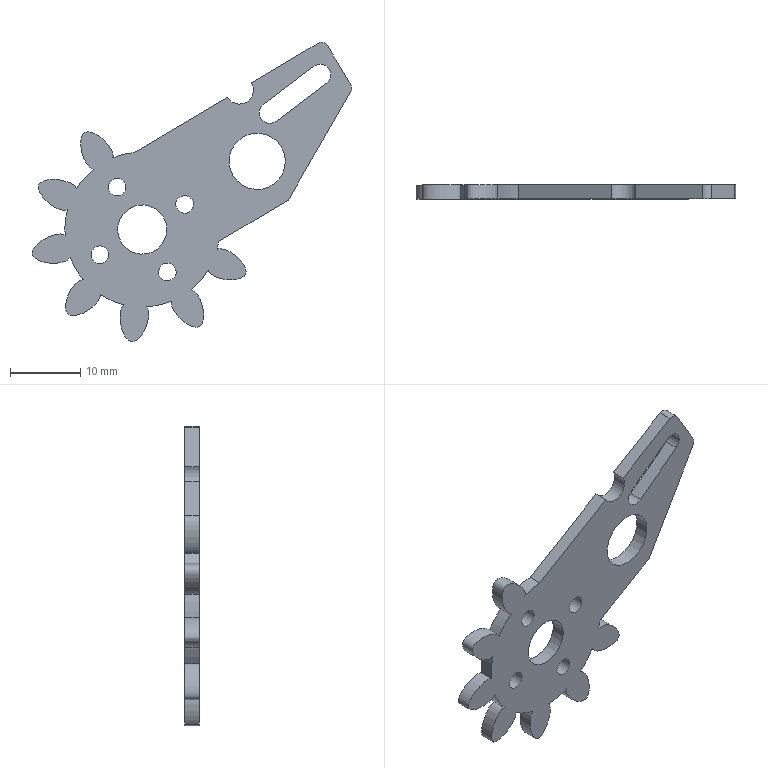Component | SolidWorks | New1Left-1 | 1 solid | 42 faces | box 45.4 x 2 x 42.54 mm | volume 1446 mm3 | cylinder 26 | plane 9 | spline 7 | commonest cylinder face diameters 2.5 x8 22 x8 3 x3 7 x2 8 x2 2 x2 4 x1
build123d program:
from build123d import *

# Parameters (mm, degrees)
SKETCH1_R           = 3.5
SKETCH1_R_2         = 4
BOSS_EXTRUDE1_DEPTH = 2
FILLET1_R           = 1
FILLET2_R           = 1
SKETCH2_R           = 1.25
CUT_EXTRUDE1_DEPTH  = 10


with BuildPart() as part:
    # Sketch1 → Boss-Extrude1 (new body)
    with BuildSketch(Plane(origin=(0, 0, 0), x_dir=(1, 0, 0), z_dir=(0, 1, 0))):
        with BuildLine():
            Line((5, 0), (0, 0))
            Line((0, 0), (0, -3))
            Line((0, -3), (0, -12))
            ThreePointArc((0, -12), (2, -14), (0, -16))
            Line((0, -16), (0, -17))
            Line((0, -17), (0, -23.51))
            Line((0, -23.51), (0, -31.417))
            ThreePointArc((0, -31.417), (-0.5475, -32.877), (-0.883, -34.4))
            add(Edge.make_bspline(
                [(-0.883, -37.6), (-2.069, -38.773), (-9.931, -36), (-2.069, -33.227), (-0.883, -34.4)],
                knots=[0, 0, 0, 0, 0.5, 1, 1, 1, 1], degree=3))
            ThreePointArc((-0.883, -37.6), (-0.4616, -39.399), (0.255, -41.102))
            add(Edge.make_bspline(
                [(2.136, -43.691), (1.866, -45.337), (-6.125, -47.715), (-1.394, -40.851), (0.255, -41.102)],
                knots=[0, 0, 0, 0, 0.5, 1, 1, 1, 1], degree=3))
            ThreePointArc((2.136, -43.691), (3.534, -44.899), (5.115, -45.856))
            add(Edge.make_bspline(
                [(8.159, -46.845), (8.908, -48.335), (3.841, -54.956), (3.633, -46.621), (5.115, -45.856)],
                knots=[0, 0, 0, 0, 0.5, 1, 1, 1, 1], degree=3))
            ThreePointArc((8.159, -46.845), (10, -47), (11.841, -46.845))
            add(Edge.make_bspline(
                [(14.885, -45.856), (16.367, -46.621), (16.159, -54.956), (11.092, -48.335), (11.841, -46.845)],
                knots=[0, 0, 0, 0, 0.5, 1, 1, 1, 1], degree=3))
            ThreePointArc((14.885, -45.856), (16.466, -44.899), (17.864, -43.691))
            add(Edge.make_bspline(
                [(19.745, -41.102), (21.394, -40.851), (26.125, -47.715), (18.134, -45.337), (17.864, -43.691)],
                knots=[0, 0, 0, 0, 0.5, 1, 1, 1, 1], degree=3))
            ThreePointArc((19.745, -41.102), (20.462, -39.399), (20.883, -37.6))
            add(Edge.make_bspline(
                [(20.883, -34.4), (22.069, -33.227), (29.931, -36), (22.069, -38.773), (20.883, -37.6)],
                knots=[0, 0, 0, 0, 0.5, 1, 1, 1, 1], degree=3))
            ThreePointArc((20.883, -34.4), (20.462, -32.601), (19.745, -30.898))
            add(Edge.make_bspline(
                [(17.864, -28.309), (18.134, -26.663), (26.125, -24.285), (21.394, -31.149), (19.745, -30.898)],
                knots=[0, 0, 0, 0, 0.5, 1, 1, 1, 1], degree=3))
            ThreePointArc((17.864, -28.309), (17.443, -27.9), (17, -27.515))
            Line((17, -27.515), (17, -21.613))
            Line((17, -21.613), (17, -16))
            Line((17, -16), (8, 0))
            Line((8, 0), (5, 0))
        make_face()
        with Locations(Location((10, -36, 0), (0, 0, 270))):
            Circle(SKETCH1_R, mode=Mode.SUBTRACT)
        with Locations(Location((10, -17, 0), (0, 0, 270))):
            Circle(SKETCH1_R_2, mode=Mode.SUBTRACT)
        with BuildLine():
            ThreePointArc((2.509, -3.167), (3.833, -1.509), (5.491, -2.833))
            Line((5.491, -2.833), (6.491, -11.778))
            ThreePointArc((6.491, -11.778), (5.167, -13.435), (3.509, -12.111))
            Line((3.509, -12.111), (2.509, -3.167))
        make_face(mode=Mode.SUBTRACT)
    extrude(amount=BOSS_EXTRUDE1_DEPTH)

    # Fillet1
    fillet1_edges = [part.edges().sort_by_distance(p)[0] for p in [
        (0, 1, 0),
    ]]
    fillet(fillet1_edges, radius=FILLET1_R)

    # Fillet2
    fillet2_edges = [part.edges().sort_by_distance(p)[0] for p in [
        (8, 1, 0),
    ]]
    fillet(fillet2_edges, radius=FILLET2_R)

    # Sketch2 → Cut-Extrude1 (cut)
    with BuildSketch(Plane(origin=(0, 2, 0), x_dir=(1, 0, 0), z_dir=(0, 1, 0))):
        with Locations(Location((10, -29, 0), (0, 0, 270))):
            Circle(SKETCH2_R)
        with Locations(Location((10, -43, 0), (0, 0, 270))):
            Circle(SKETCH2_R)
        with Locations(Location((17, -36, 0), (0, 0, 270))):
            Circle(SKETCH2_R)
        with Locations(Location((3, -36, 0), (0, 0, 270))):
            Circle(SKETCH2_R)
    extrude(amount=-CUT_EXTRUDE1_DEPTH, mode=Mode.SUBTRACT)


solid = part.part

# Placed as in the assembly
solid = solid.moved(Location((35.043, 23.961, 80.978), (180, -59.299, 0)))